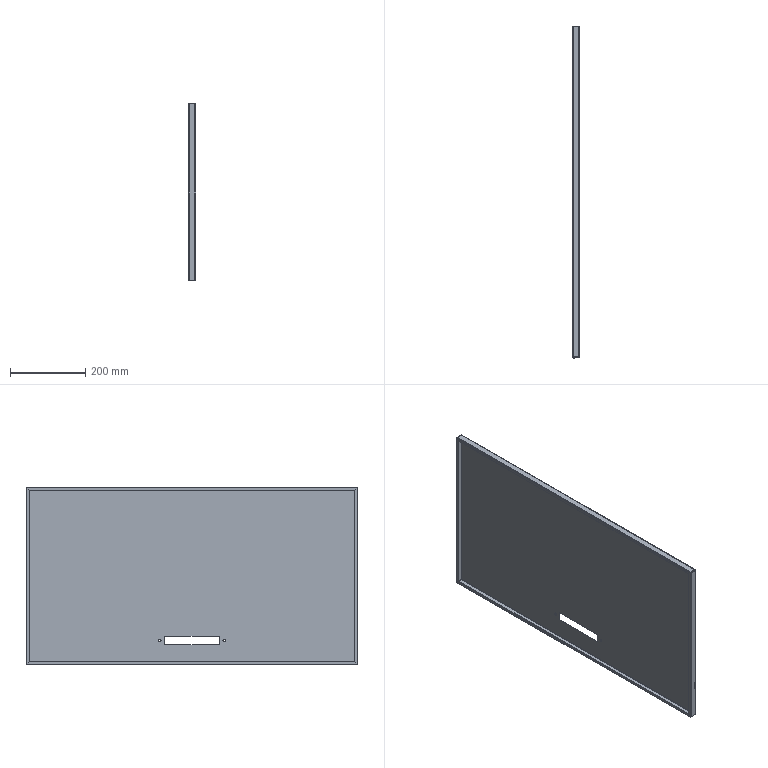Component | SolidWorks | FrontLeftDoor-1_FrontLeftDoorPanel100-1 | 1 solid | 78 faces | volume 714055 mm3 | plane 42 | cylinder 20 | spline 16 | commonest cylinder face diameters 4.473 x8 1.473 x8 6 x4